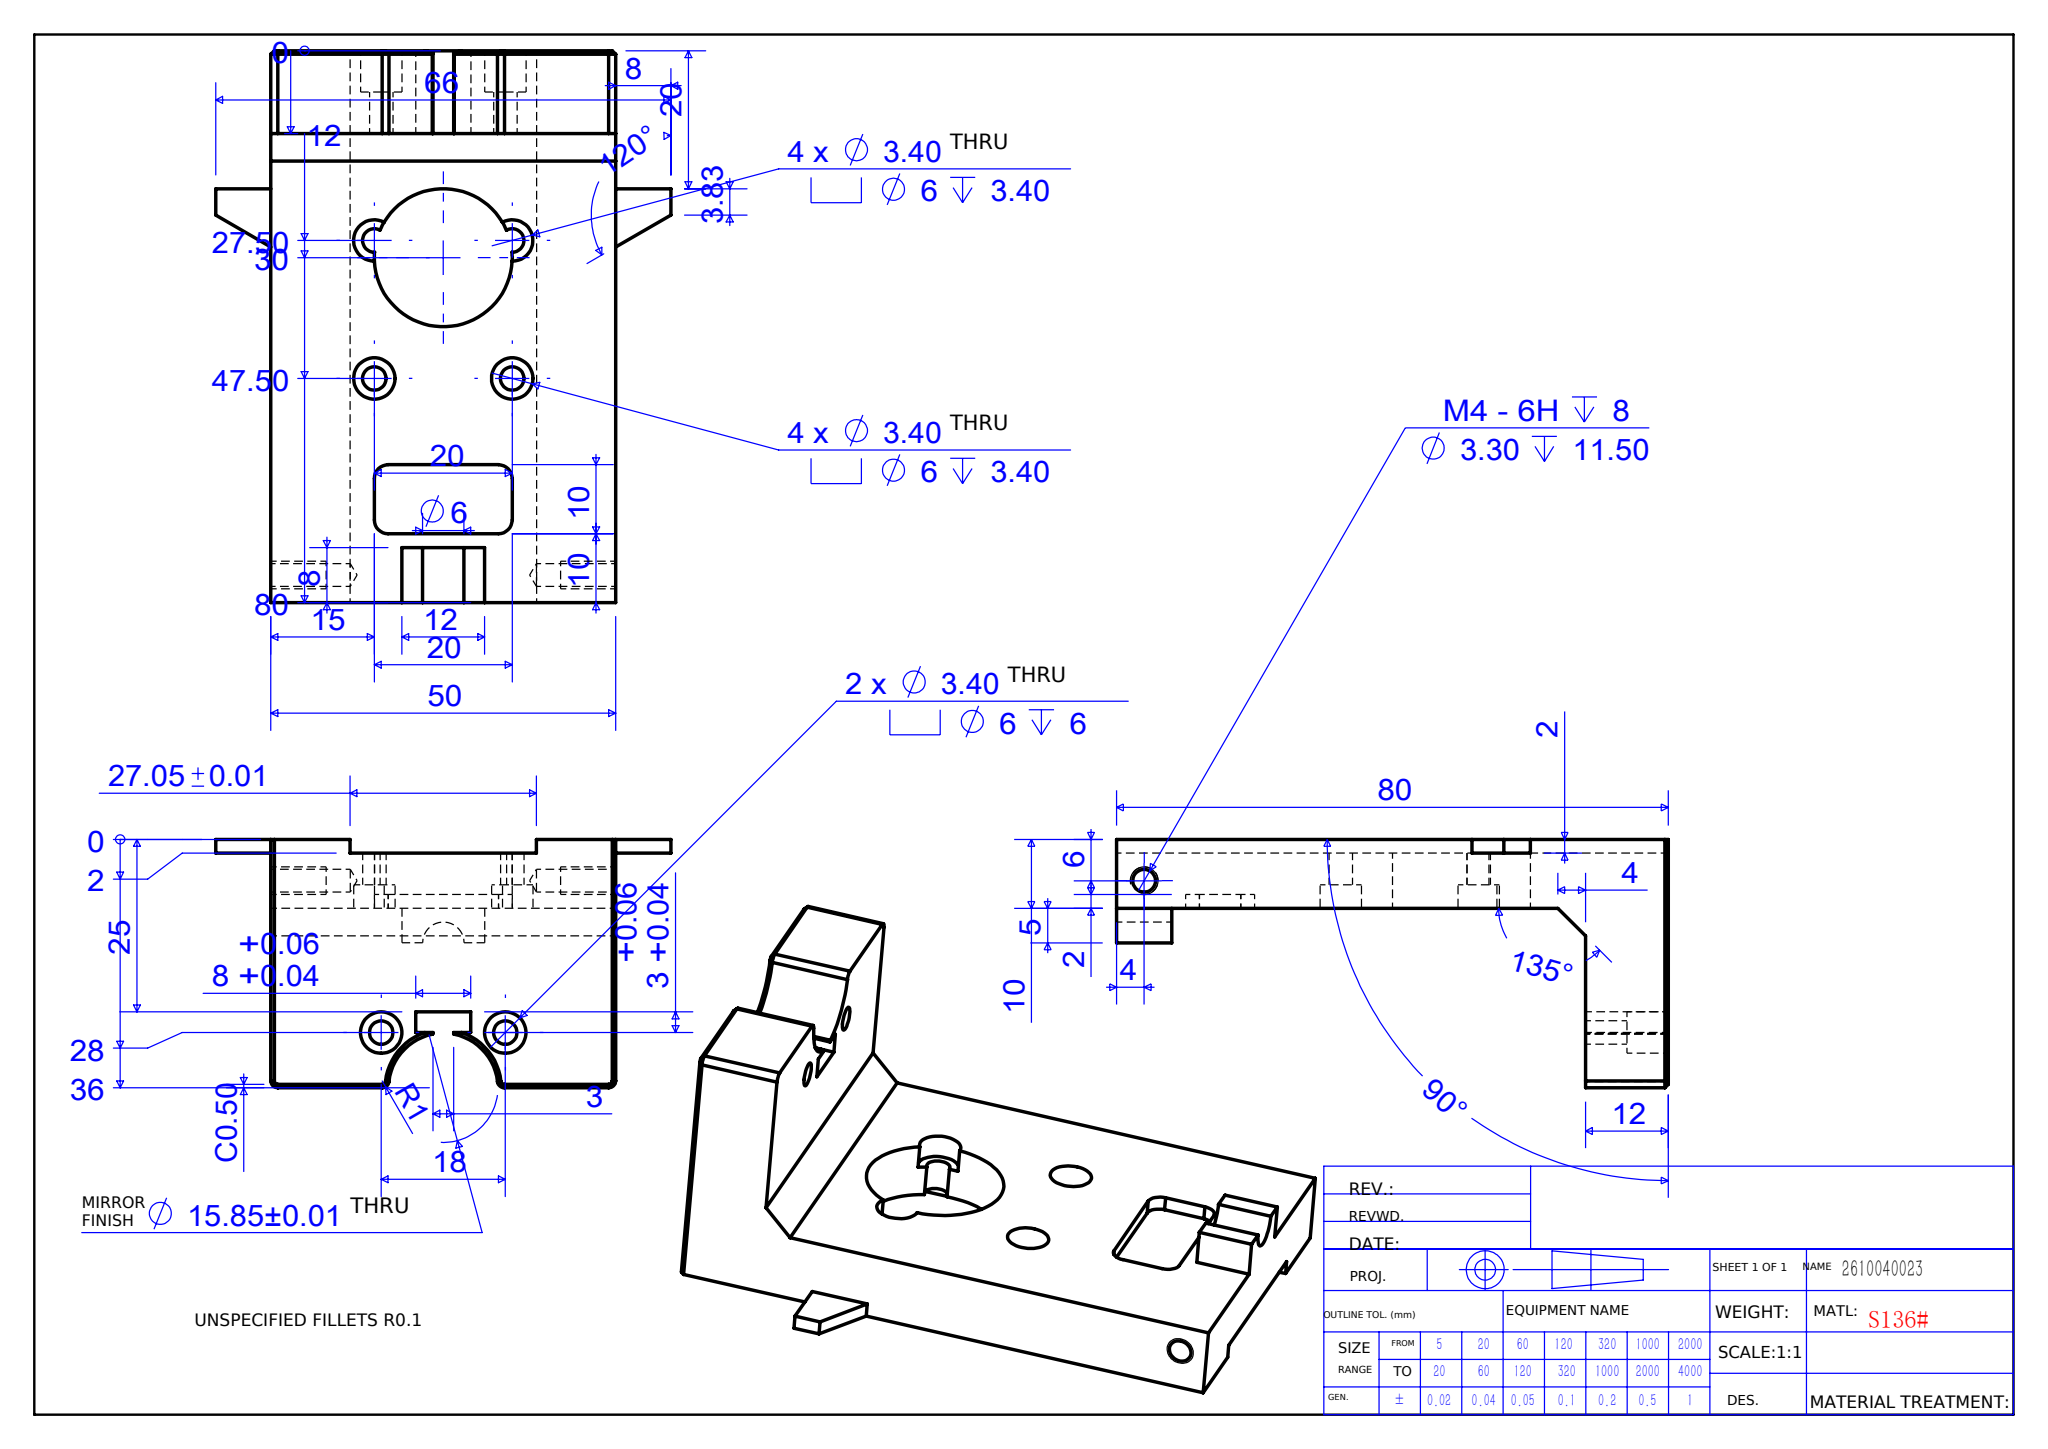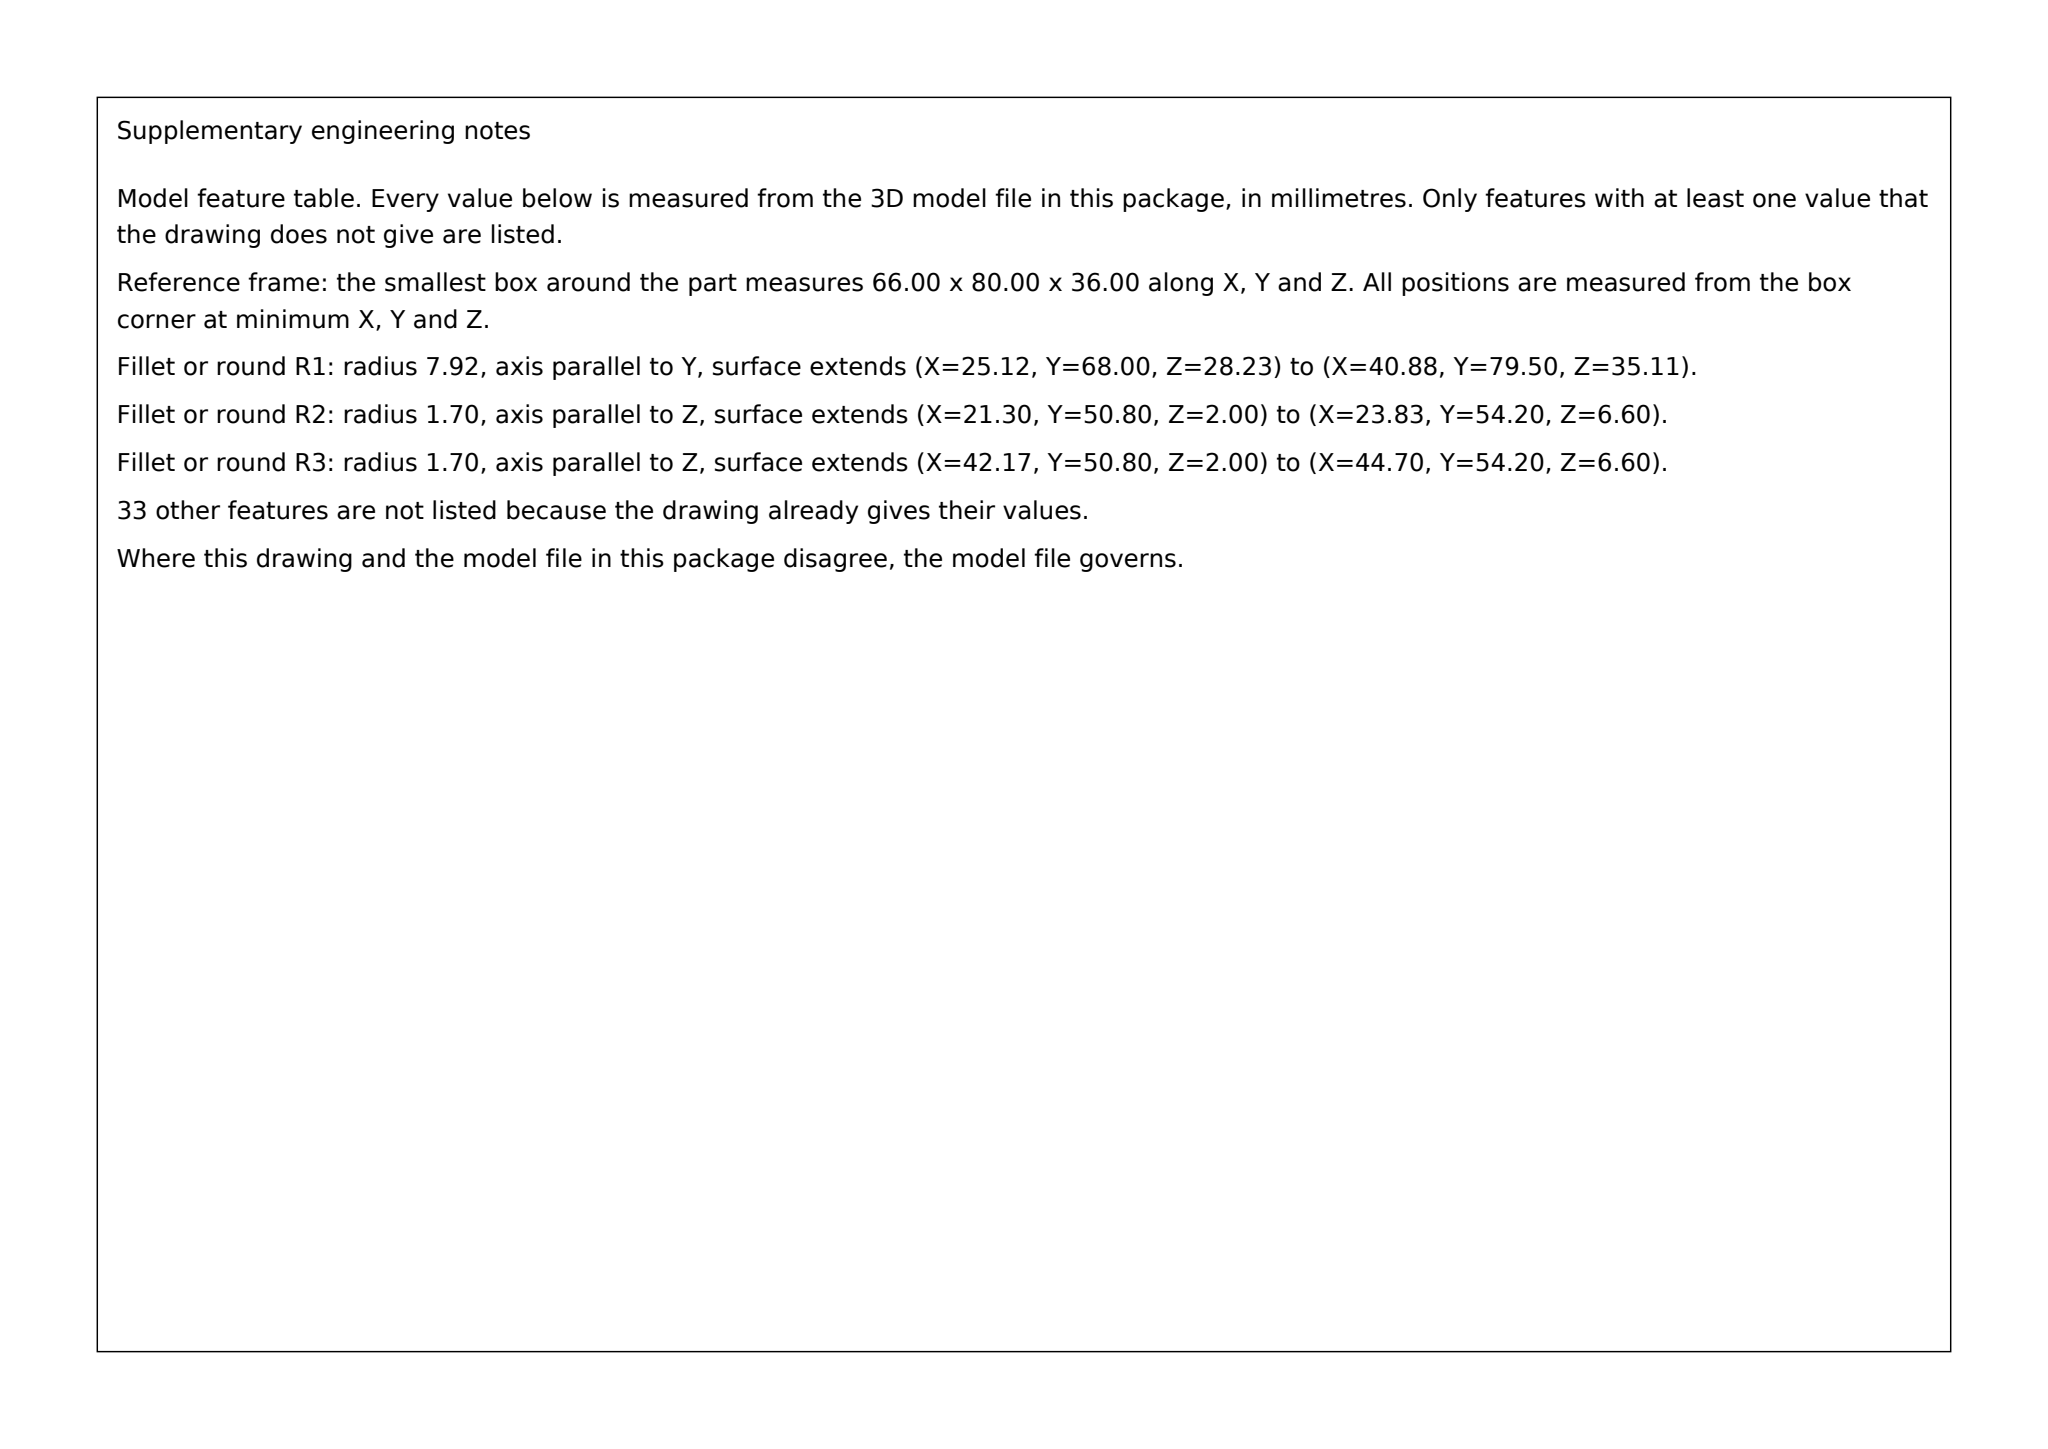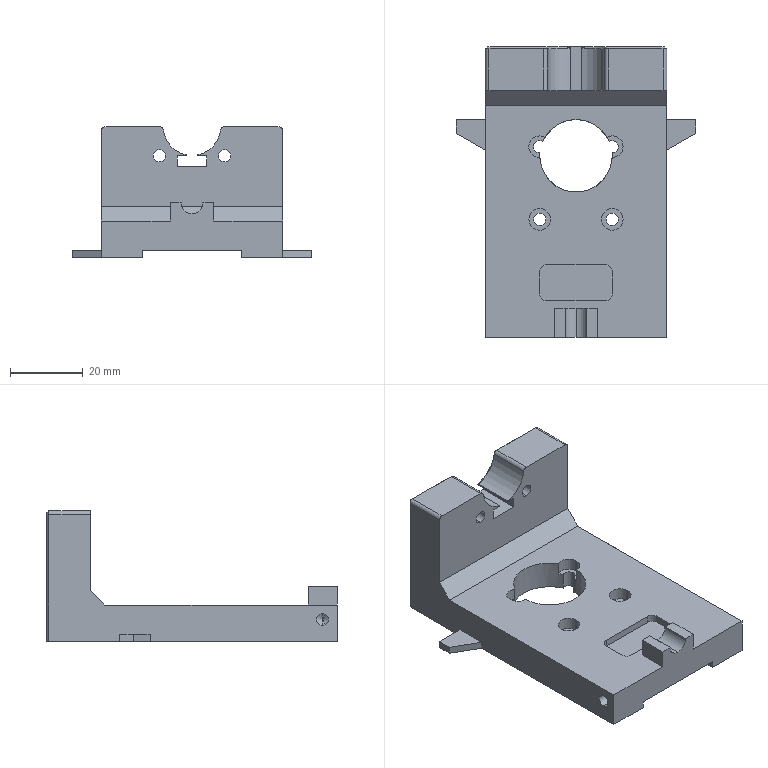Part | SolidWorks | mm | material S136# | 1 solid | 103 faces | box 66 x 80 x 36 mm | volume 46734 mm3 | plane 49 | cylinder 44 | cone 10 | commonest cylinder face diameters 6 x13 3.4 x11 3.3 x4 20 x4 2 x4 4 x4 15.85 x2 0.2 x2